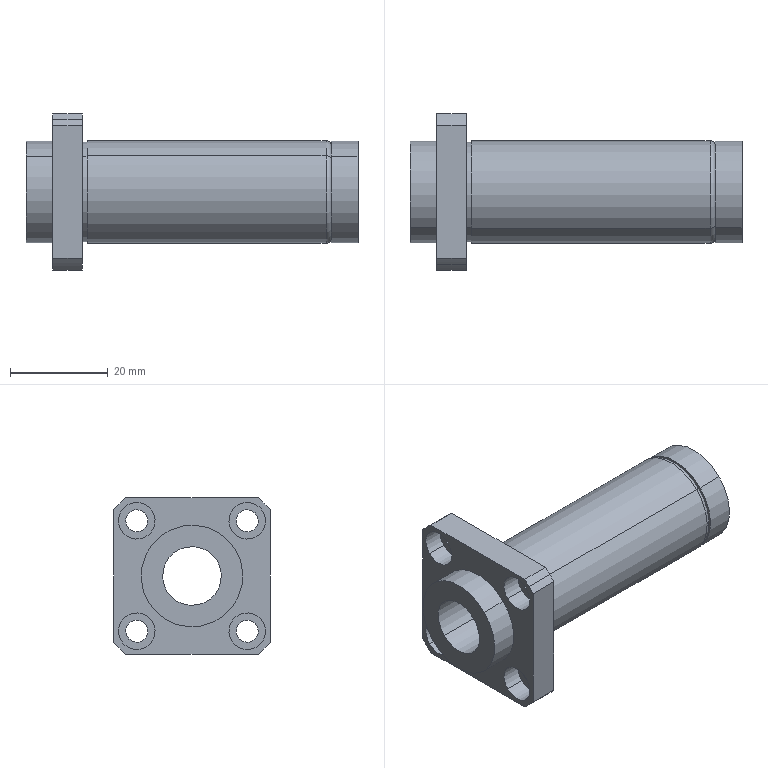Component | SolidWorks | LHFRW_MX12-1 | 1 solid | 47 faces | volume 18910 mm3 | cylinder 31 | plane 14 | torus 2 | commonest cylinder face diameters 4.5 x8 7.5 x8 42 x5 20.8 x4 20.4 x2 21 x2 12 x2